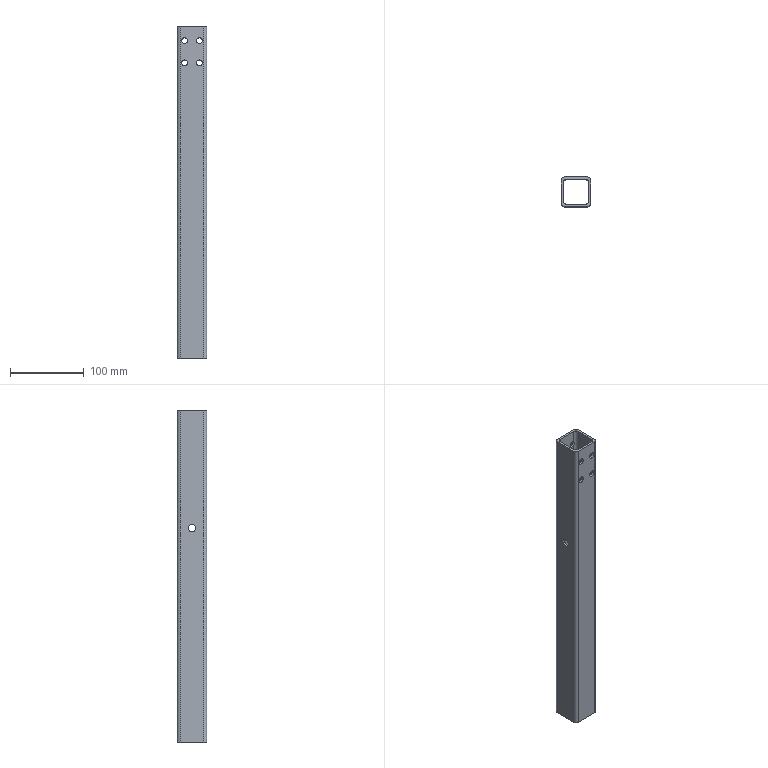Component | NX | TOP_ROD_2_2 | 1 solid | 28 faces | volume 198122 mm3 | cylinder 18 | plane 10 | commonest cylinder face diameters 8 x16 10 x2